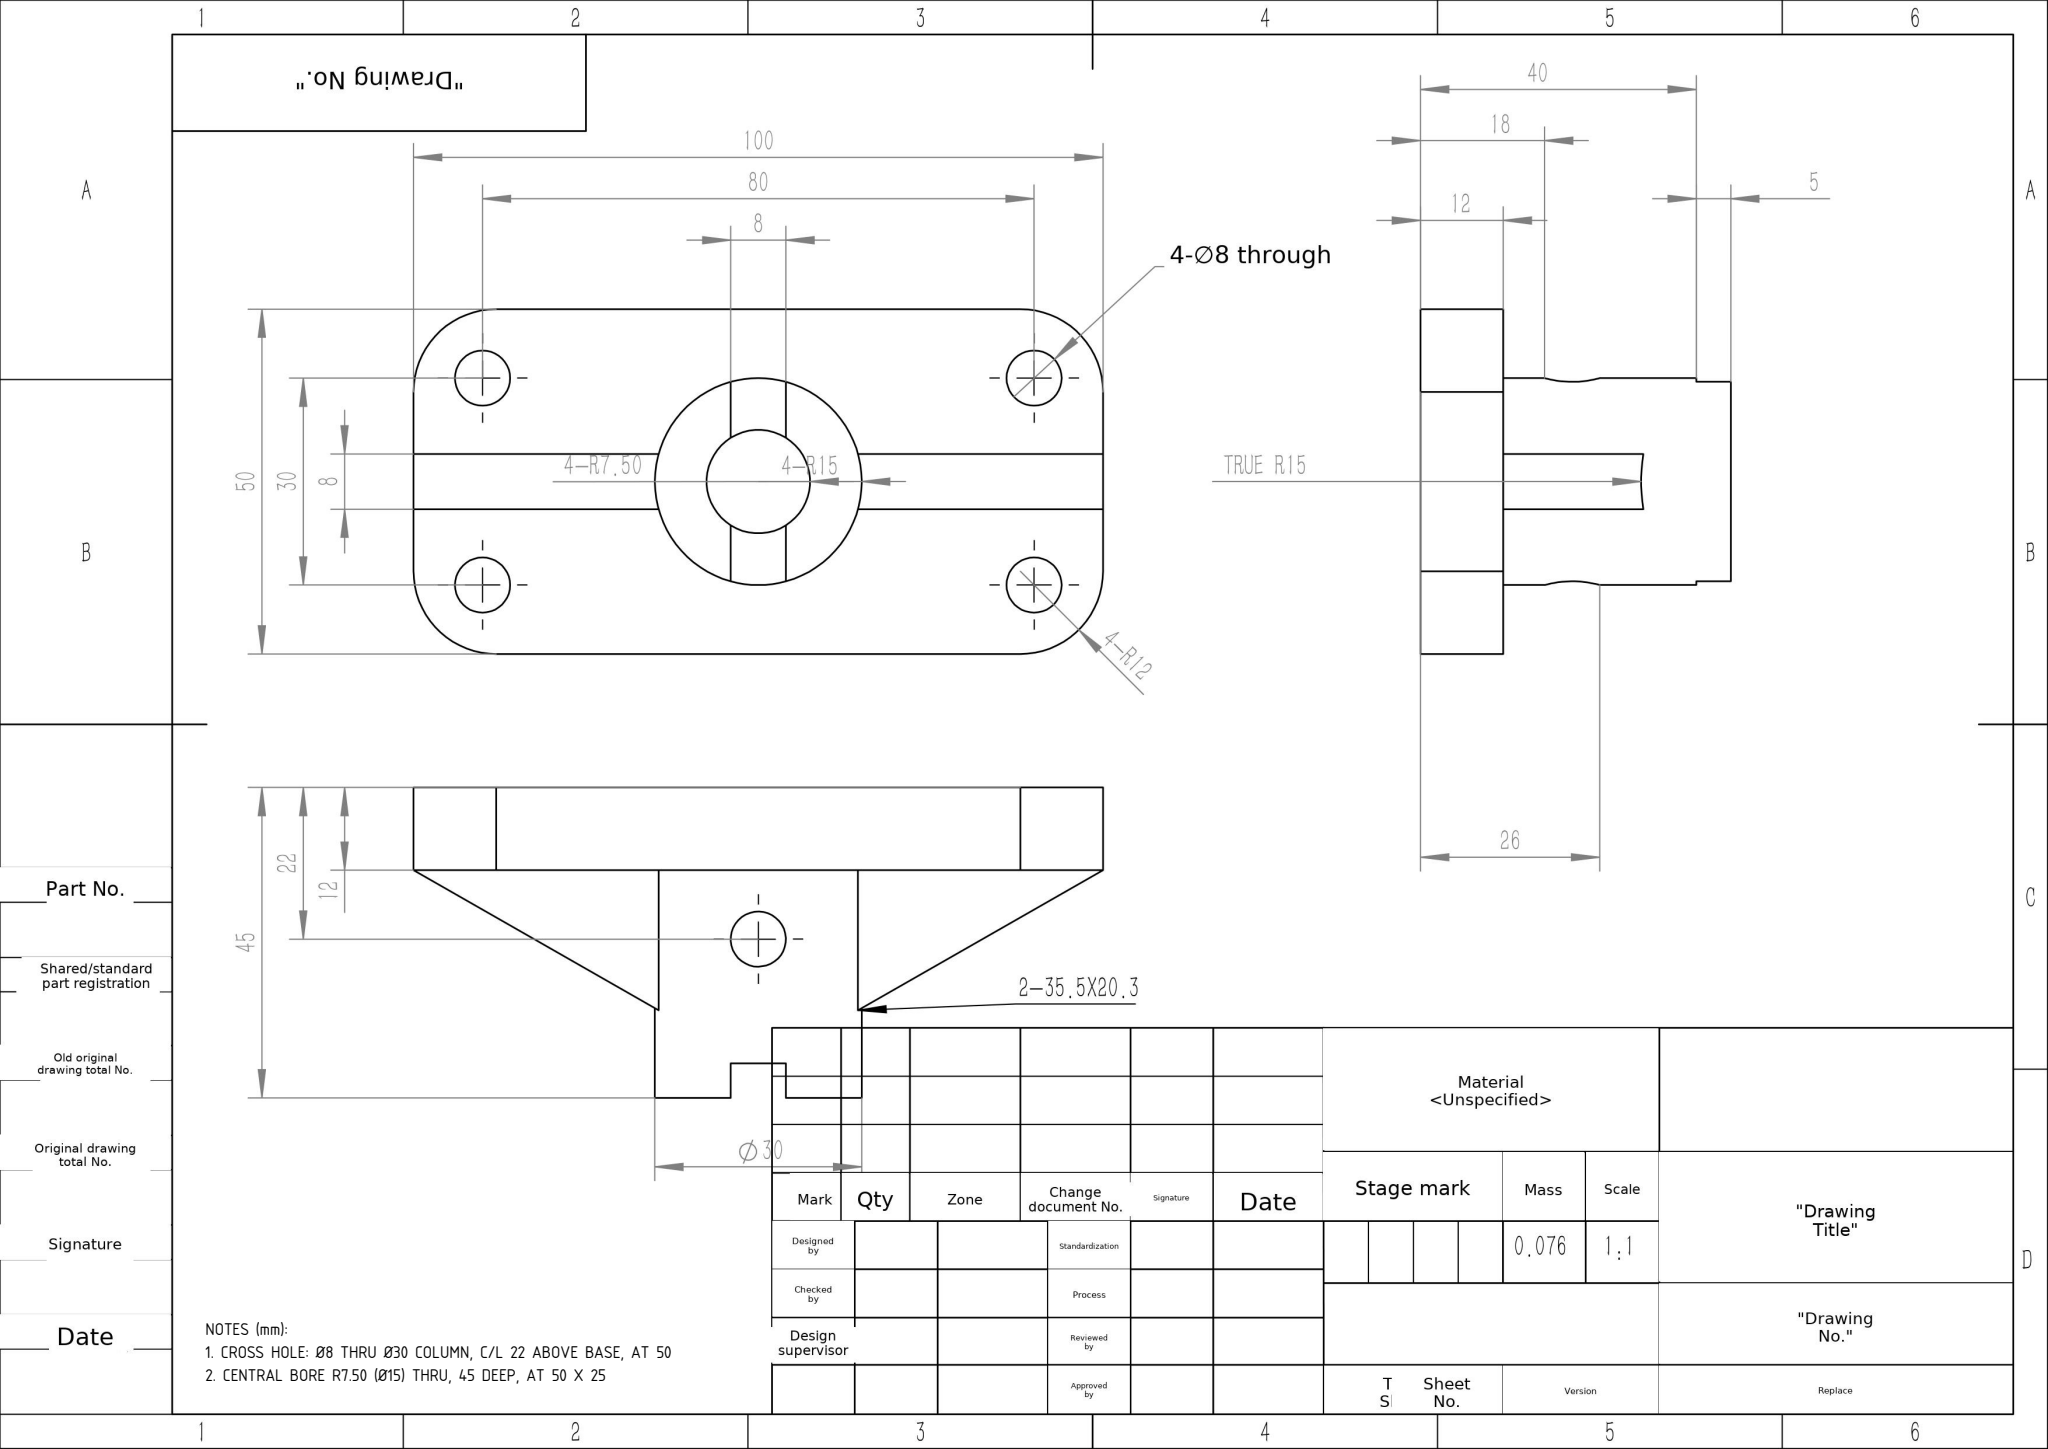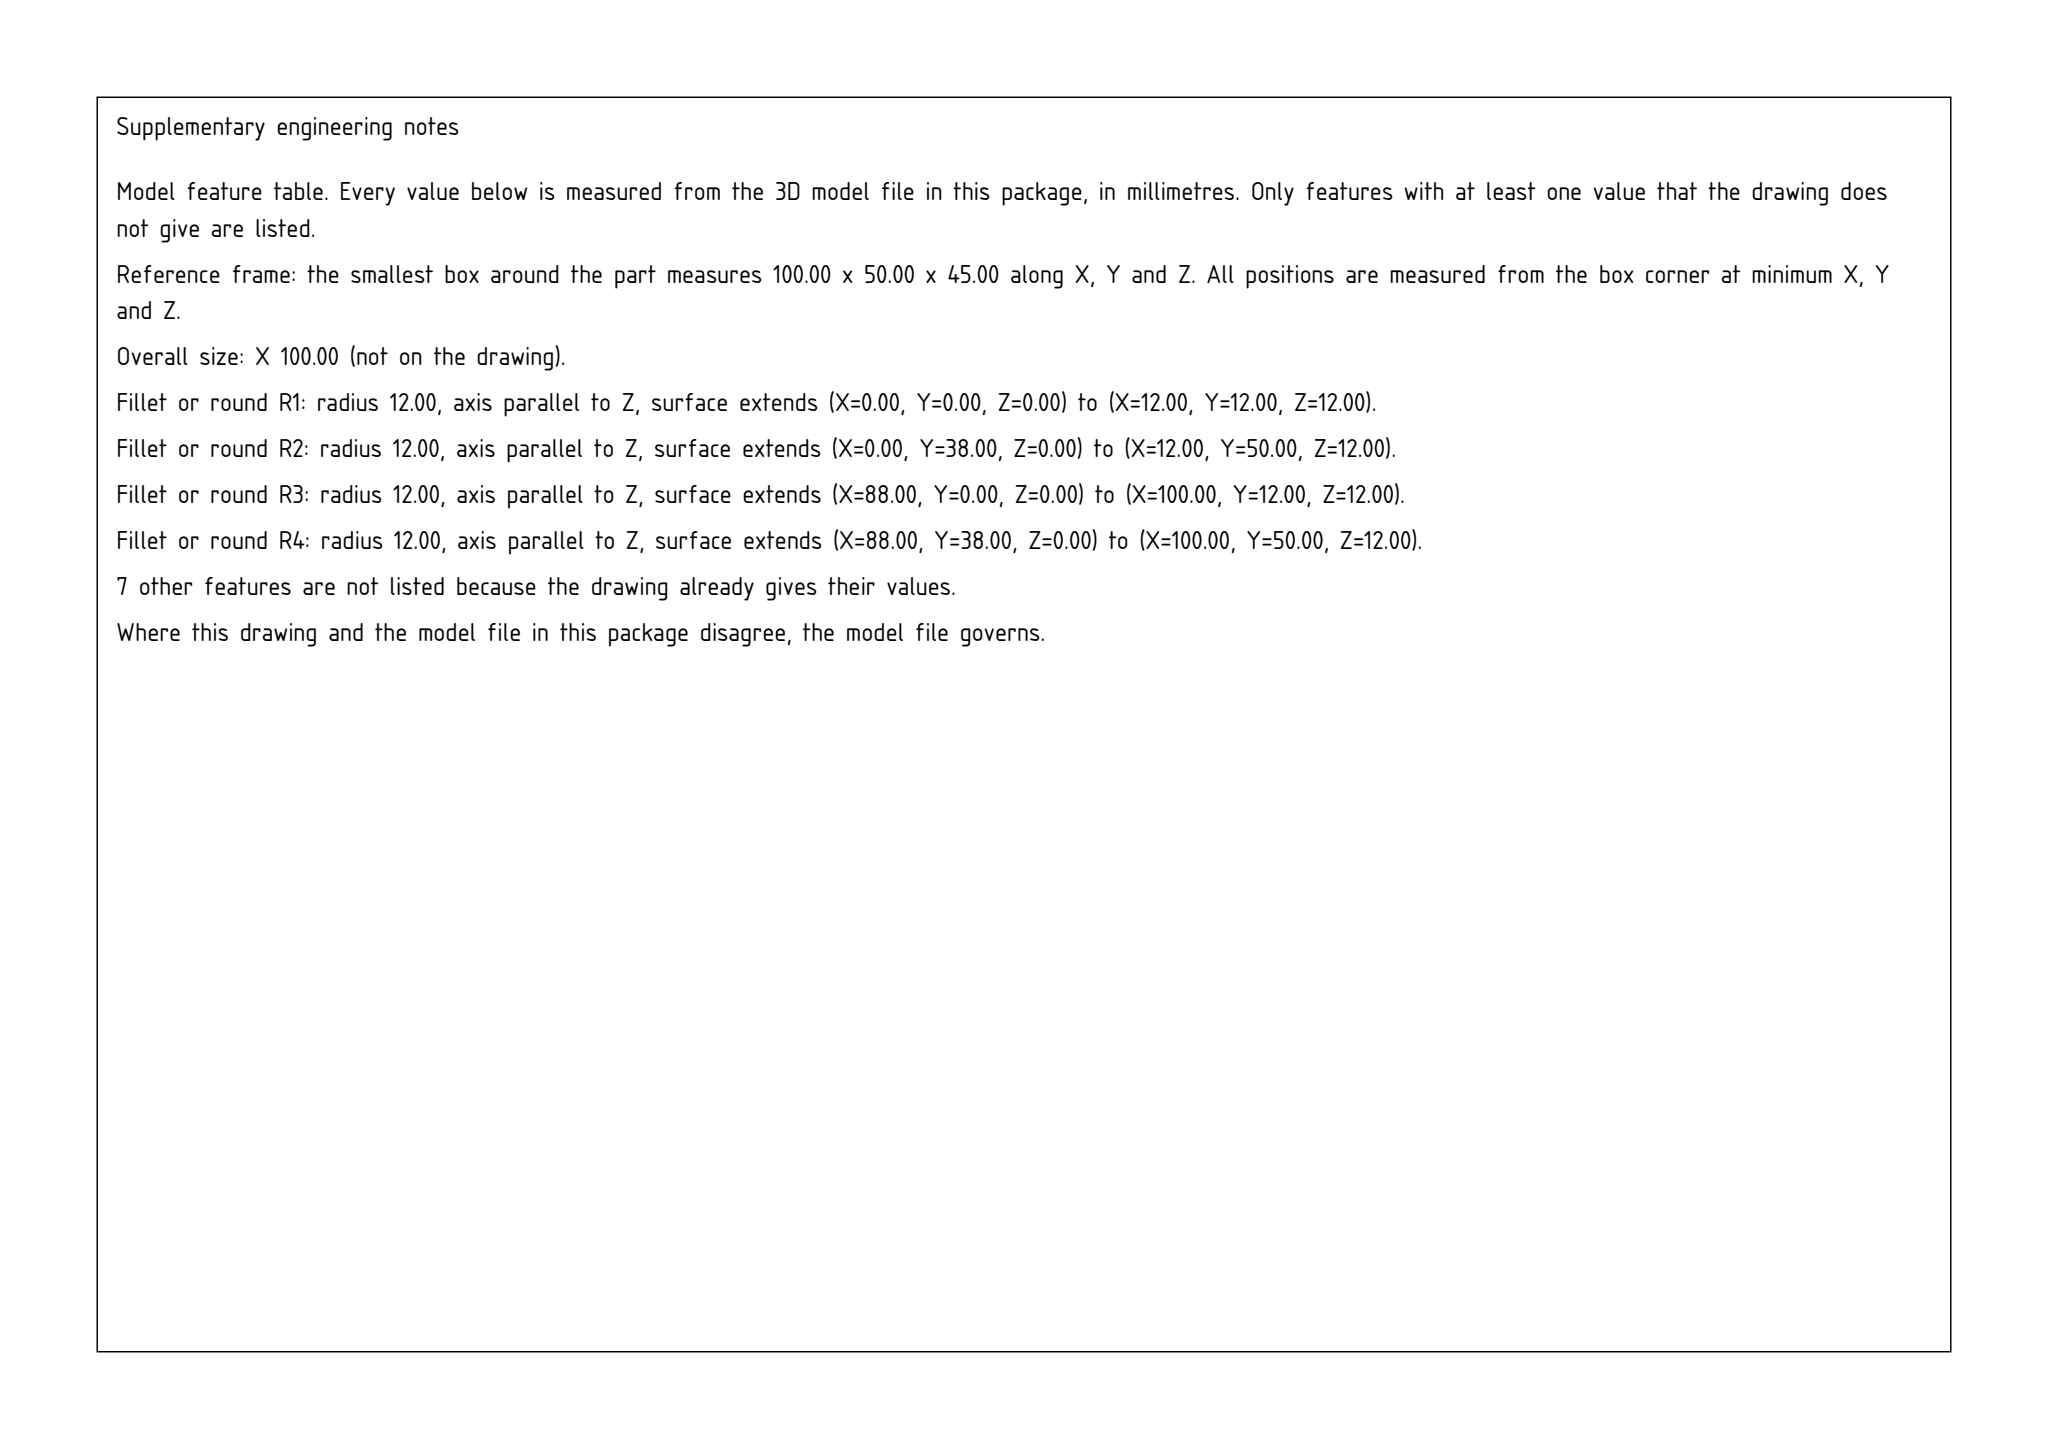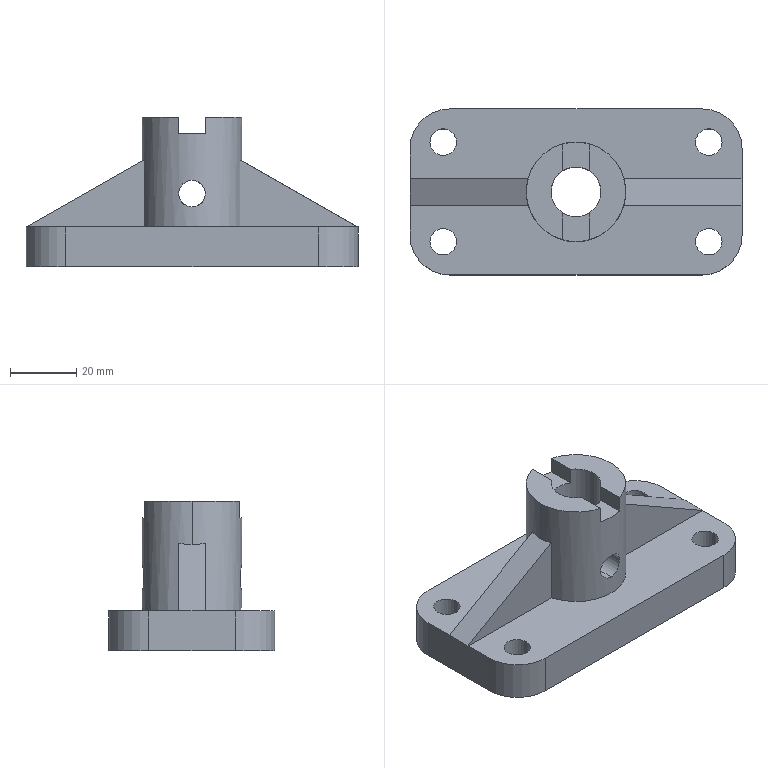Part | SolidWorks | mm | 1 solid | 41 faces | box 100 x 50 x 45 mm | volume 75752 mm3 | plane 21 | cylinder 20 | commonest cylinder face diameters 8 x12 24 x4 15 x2 30 x2
Drawing notes:
CROSS HOLE: Ø8 THRU Ø30 COLUMN, C/L 22 ABOVE BASE, AT 50 | from the solid: cylinder dia 8.0 axis y at x=50.0, z=22.0, length 8.66 (thru Ø30 boss)
CENTRAL BORE R7.50 (Ø15) THRU, 45 DEEP, AT 50 X 25 | from the solid: cylinder dia 15.0 axis z at x=50.0, y=25.0, length 45.0 = full bbox height